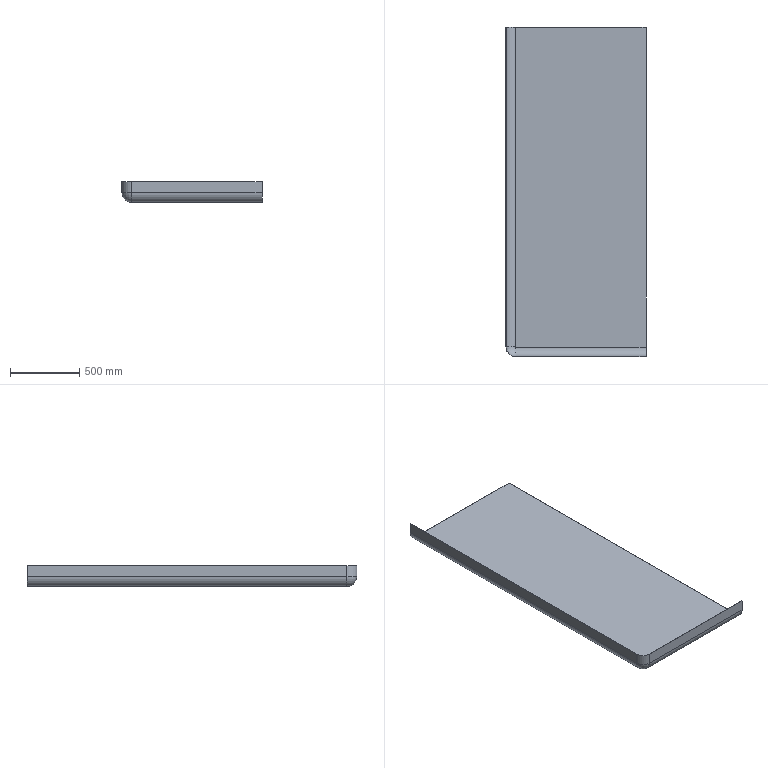Component | SolidWorks | C-SideAluminumHousingAssembly-1_C-SideAluminumCasing2-1 | 1 solid | 21 faces | box 1009.5 x 2375.5 x 149.5 mm | volume 8369304 mm3 | plane 13 | cylinder 6 | torus 2 | commonest cylinder face diameters 139 x2 133 x2 141 x1 135 x1
STEP:
#1=CARTESIAN_POINT('',(-0.2362,0.,-0.1181));
#2=VERTEX_POINT('',#1);
#3=CARTESIAN_POINT('',(-0.2362,0.,0.));
#4=VERTEX_POINT('',#3);
#5=CARTESIAN_POINT('',(-0.2362,0.,0.));
#6=DIRECTION('',(0.,0.,1.));
#7=VECTOR('',#6,39.37);
#8=LINE('',#5,#7);
#9=EDGE_CURVE('',#2,#4,#8,.T.);
#10=ORIENTED_EDGE('',*,*,#9,.F.);
#11=CARTESIAN_POINT('',(-0.2362,90.787,-0.1181));
#12=VERTEX_POINT('',#11);
#13=CARTESIAN_POINT('',(-0.2362,0.,-0.1181));
#14=DIRECTION('',(0.,1.,0.));
#15=VECTOR('',#14,39.37);
#16=LINE('',#13,#15);
#17=EDGE_CURVE('',#2,#12,#16,.T.);
#18=ORIENTED_EDGE('',*,*,#17,.T.);
#19=CARTESIAN_POINT('',(-0.2362,90.787,0.));
#20=VERTEX_POINT('',#19);
#21=CARTESIAN_POINT('',(-0.2362,90.787,0.));
#22=DIRECTION('',(0.,0.,1.));
#23=VECTOR('',#22,39.37);
#24=LINE('',#21,#23);
#25=EDGE_CURVE('',#12,#20,#24,.T.);
#26=ORIENTED_EDGE('',*,*,#25,.T.);
#27=CARTESIAN_POINT('',(-0.2362,0.,0.));
#28=DIRECTION('',(0.,1.,0.));
#29=VECTOR('',#28,39.37);
#30=LINE('',#27,#29);
#31=EDGE_CURVE('',#4,#20,#30,.T.);
#32=ORIENTED_EDGE('',*,*,#31,.F.);
#33=EDGE_LOOP('',(#10,#18,#26,#32));
#34=FACE_OUTER_BOUND('',#33,.T.);
#35=CARTESIAN_POINT('',(-0.2362,0.,0.));
#36=DIRECTION('',(-1.,0.,0.));
#37=DIRECTION('',(0.,1.,0.));
#38=AXIS2_PLACEMENT_3D('',#35,#36,#37);
#39=PLANE('',#38);
#40=ADVANCED_FACE('',(#34),#39,.F.);
#41=ORIENTED_EDGE('',*,*,#25,.F.);
#42=CARTESIAN_POINT('',(-37.244,90.787,-0.1181));
#43=VERTEX_POINT('',#42);
#44=CARTESIAN_POINT('',(-37.244,90.787,-0.1181));
#45=DIRECTION('',(-1.,0.,0.));
#46=VECTOR('',#45,39.37);
#47=LINE('',#44,#46);
#48=EDGE_CURVE('',#12,#43,#47,.T.);
#49=ORIENTED_EDGE('',*,*,#48,.T.);
#50=CARTESIAN_POINT('',(-37.244,90.787,0.));
#51=VERTEX_POINT('',#50);
#52=CARTESIAN_POINT('',(-37.244,90.787,0.));
#53=DIRECTION('',(0.,0.,1.));
#54=VECTOR('',#53,39.37);
#55=LINE('',#52,#54);
#56=EDGE_CURVE('',#43,#51,#55,.T.);
#57=ORIENTED_EDGE('',*,*,#56,.T.);
#58=CARTESIAN_POINT('',(-37.244,90.787,0.));
#59=DIRECTION('',(-1.,0.,0.));
#60=VECTOR('',#59,39.37);
#61=LINE('',#58,#60);
#62=EDGE_CURVE('',#20,#51,#61,.T.);
#63=ORIENTED_EDGE('',*,*,#62,.F.);
#64=EDGE_LOOP('',(#41,#49,#57,#63));
#65=FACE_OUTER_BOUND('',#64,.T.);
#66=CARTESIAN_POINT('',(-37.244,90.787,0.));
#67=DIRECTION('',(0.,-1.,0.));
#68=DIRECTION('',(-1.,0.,0.));
#69=AXIS2_PLACEMENT_3D('',#66,#67,#68);
#70=PLANE('',#69);
#71=ADVANCED_FACE('',(#65),#70,.F.);
#72=CARTESIAN_POINT('',(-37.244,0.03937,0.));
#73=VERTEX_POINT('',#72);
#74=CARTESIAN_POINT('',(-37.244,0.,0.));
#75=DIRECTION('',(0.,-1.,0.));
#76=VECTOR('',#75,39.37);
#77=LINE('',#74,#76);
#78=EDGE_CURVE('',#51,#73,#77,.T.);
#79=ORIENTED_EDGE('',*,*,#78,.T.);
#80=CARTESIAN_POINT('',(-37.205,0.,0.));
#81=VERTEX_POINT('',#80);
#82=CARTESIAN_POINT('',(-37.205,0.03937,0.));
#83=DIRECTION('',(0.,0.,1.));
#84=DIRECTION('',(-1.,0.,0.));
#85=AXIS2_PLACEMENT_3D('',#82,#83,#84);
#86=CIRCLE('',#85,0.03937);
#87=EDGE_CURVE('',#73,#81,#86,.T.);
#88=ORIENTED_EDGE('',*,*,#87,.T.);
#89=CARTESIAN_POINT('',(-37.244,0.,0.));
#90=DIRECTION('',(1.,0.,0.));
#91=VECTOR('',#90,39.37);
#92=LINE('',#89,#91);
#93=EDGE_CURVE('',#81,#4,#92,.T.);
#94=ORIENTED_EDGE('',*,*,#93,.T.);
#95=ORIENTED_EDGE('',*,*,#31,.T.);
#96=ORIENTED_EDGE('',*,*,#62,.T.);
#97=EDGE_LOOP('',(#79,#88,#94,#95,#96));
#98=FACE_OUTER_BOUND('',#97,.T.);
#99=CARTESIAN_POINT('',(-37.244,0.,0.));
#100=DIRECTION('',(0.,0.,-1.));
#101=DIRECTION('',(-1.,0.,0.));
#102=AXIS2_PLACEMENT_3D('',#99,#100,#101);
#103=PLANE('',#102);
#104=ADVANCED_FACE('',(#98),#103,.F.);
#105=CARTESIAN_POINT('',(-37.205,0.,-0.1181));
#106=VERTEX_POINT('',#105);
#107=CARTESIAN_POINT('',(-37.244,0.,-0.1181));
#108=DIRECTION('',(1.,0.,0.));
#109=VECTOR('',#108,39.37);
#110=LINE('',#107,#109);
#111=EDGE_CURVE('',#106,#2,#110,.T.);
#112=ORIENTED_EDGE('',*,*,#111,.F.);
#113=CARTESIAN_POINT('',(-37.244,0.03937,-0.1181));
#114=VERTEX_POINT('',#113);
#115=CARTESIAN_POINT('',(-37.205,0.03937,-0.1181));
#116=DIRECTION('',(0.,0.,-1.));
#117=DIRECTION('',(-1.,0.,0.));
#118=AXIS2_PLACEMENT_3D('',#115,#116,#117);
#119=CIRCLE('',#118,0.03937);
#120=EDGE_CURVE('',#106,#114,#119,.T.);
#121=ORIENTED_EDGE('',*,*,#120,.T.);
#122=CARTESIAN_POINT('',(-37.244,0.,-0.1181));
#123=DIRECTION('',(0.,-1.,0.));
#124=VECTOR('',#123,39.37);
#125=LINE('',#122,#124);
#126=EDGE_CURVE('',#43,#114,#125,.T.);
#127=ORIENTED_EDGE('',*,*,#126,.F.);
#128=ORIENTED_EDGE('',*,*,#48,.F.);
#129=ORIENTED_EDGE('',*,*,#17,.F.);
#130=EDGE_LOOP('',(#112,#121,#127,#128,#129));
#131=FACE_OUTER_BOUND('',#130,.T.);
#132=CARTESIAN_POINT('',(-37.244,0.,-0.1181));
#133=DIRECTION('',(0.,0.,-1.));
#134=DIRECTION('',(-1.,0.,0.));
#135=AXIS2_PLACEMENT_3D('',#132,#133,#134);
#136=PLANE('',#135);
#137=ADVANCED_FACE('',(#131),#136,.T.);
#138=CARTESIAN_POINT('',(-0.2362,-2.618,2.618));
#139=VERTEX_POINT('',#138);
#140=CARTESIAN_POINT('',(-0.2362,0.,2.618));
#141=DIRECTION('',(1.,0.,0.));
#142=DIRECTION('',(0.,0.,-1.));
#143=AXIS2_PLACEMENT_3D('',#140,#141,#142);
#144=CIRCLE('',#143,2.618);
#145=EDGE_CURVE('',#139,#4,#144,.T.);
#146=ORIENTED_EDGE('',*,*,#145,.F.);
#147=CARTESIAN_POINT('',(-0.2362,-2.736,2.618));
#148=VERTEX_POINT('',#147);
#149=CARTESIAN_POINT('',(-0.2362,-2.618,2.618));
#150=DIRECTION('',(0.,-1.,-0.));
#151=VECTOR('',#150,39.37);
#152=LINE('',#149,#151);
#153=EDGE_CURVE('',#139,#148,#152,.T.);
#154=ORIENTED_EDGE('',*,*,#153,.T.);
#155=CARTESIAN_POINT('',(-0.2362,0.,2.618));
#156=DIRECTION('',(1.,0.,0.));
#157=DIRECTION('',(0.,0.,-1.));
#158=AXIS2_PLACEMENT_3D('',#155,#156,#157);
#159=CIRCLE('',#158,2.736);
#160=EDGE_CURVE('',#148,#2,#159,.T.);
#161=ORIENTED_EDGE('',*,*,#160,.T.);
#162=ORIENTED_EDGE('',*,*,#9,.T.);
#163=EDGE_LOOP('',(#146,#154,#161,#162));
#164=FACE_OUTER_BOUND('',#163,.T.);
#165=CARTESIAN_POINT('',(-0.2362,0.,2.618));
#166=DIRECTION('',(-1.,0.,0.));
#167=DIRECTION('',(0.,0.,1.));
#168=AXIS2_PLACEMENT_3D('',#165,#166,#167);
#169=PLANE('',#168);
#170=ADVANCED_FACE('',(#164),#169,.F.);
#171=ORIENTED_EDGE('',*,*,#111,.T.);
#172=ORIENTED_EDGE('',*,*,#160,.F.);
#173=CARTESIAN_POINT('',(-37.205,-2.736,2.618));
#174=VERTEX_POINT('',#173);
#175=CARTESIAN_POINT('',(-37.205,-2.736,2.618));
#176=DIRECTION('',(-1.,0.,0.));
#177=VECTOR('',#176,39.37);
#178=LINE('',#175,#177);
#179=EDGE_CURVE('',#148,#174,#178,.T.);
#180=ORIENTED_EDGE('',*,*,#179,.T.);
#181=CARTESIAN_POINT('',(-37.205,0.,2.618));
#182=DIRECTION('',(-1.,0.,0.));
#183=DIRECTION('',(0.,0.,-1.));
#184=AXIS2_PLACEMENT_3D('',#181,#182,#183);
#185=CIRCLE('',#184,2.736);
#186=EDGE_CURVE('',#106,#174,#185,.T.);
#187=ORIENTED_EDGE('',*,*,#186,.F.);
#188=EDGE_LOOP('',(#171,#172,#180,#187));
#189=FACE_OUTER_BOUND('',#188,.T.);
#190=CARTESIAN_POINT('',(-0.2362,0.,2.618));
#191=DIRECTION('',(1.,0.,0.));
#192=DIRECTION('',(0.,-1.,-0.));
#193=AXIS2_PLACEMENT_3D('',#190,#191,#192);
#194=CYLINDRICAL_SURFACE('',#193,2.736);
#195=ADVANCED_FACE('',(#189),#194,.T.);
#196=ORIENTED_EDGE('',*,*,#93,.F.);
#197=CARTESIAN_POINT('',(-37.205,-2.618,2.618));
#198=VERTEX_POINT('',#197);
#199=CARTESIAN_POINT('',(-37.205,0.,2.618));
#200=DIRECTION('',(-1.,0.,0.));
#201=DIRECTION('',(0.,0.,-1.));
#202=AXIS2_PLACEMENT_3D('',#199,#200,#201);
#203=CIRCLE('',#202,2.618);
#204=EDGE_CURVE('',#81,#198,#203,.T.);
#205=ORIENTED_EDGE('',*,*,#204,.T.);
#206=CARTESIAN_POINT('',(-37.205,-2.618,2.618));
#207=DIRECTION('',(1.,0.,0.));
#208=VECTOR('',#207,39.37);
#209=LINE('',#206,#208);
#210=EDGE_CURVE('',#198,#139,#209,.T.);
#211=ORIENTED_EDGE('',*,*,#210,.T.);
#212=ORIENTED_EDGE('',*,*,#145,.T.);
#213=EDGE_LOOP('',(#196,#205,#211,#212));
#214=FACE_OUTER_BOUND('',#213,.T.);
#215=CARTESIAN_POINT('',(-0.2362,0.,2.618));
#216=DIRECTION('',(1.,0.,0.));
#217=DIRECTION('',(0.,-1.,-0.));
#218=AXIS2_PLACEMENT_3D('',#215,#216,#217);
#219=CYLINDRICAL_SURFACE('',#218,2.618);
#220=ADVANCED_FACE('',(#214),#219,.F.);
#221=ORIENTED_EDGE('',*,*,#153,.F.);
#222=CARTESIAN_POINT('',(-0.2362,-2.618,5.768));
#223=VERTEX_POINT('',#222);
#224=CARTESIAN_POINT('',(-0.2362,-2.618,5.768));
#225=DIRECTION('',(0.,-0.,1.));
#226=VECTOR('',#225,39.37);
#227=LINE('',#224,#226);
#228=EDGE_CURVE('',#139,#223,#227,.T.);
#229=ORIENTED_EDGE('',*,*,#228,.T.);
#230=CARTESIAN_POINT('',(-0.2362,-2.736,5.768));
#231=VERTEX_POINT('',#230);
#232=CARTESIAN_POINT('',(-0.2362,-2.736,5.768));
#233=DIRECTION('',(0.,1.,0.));
#234=VECTOR('',#233,39.37);
#235=LINE('',#232,#234);
#236=EDGE_CURVE('',#231,#223,#235,.T.);
#237=ORIENTED_EDGE('',*,*,#236,.F.);
#238=CARTESIAN_POINT('',(-0.2362,-2.736,-0.));
#239=DIRECTION('',(0.,-0.,1.));
#240=VECTOR('',#239,39.37);
#241=LINE('',#238,#240);
#242=EDGE_CURVE('',#148,#231,#241,.T.);
#243=ORIENTED_EDGE('',*,*,#242,.F.);
#244=EDGE_LOOP('',(#221,#229,#237,#243));
#245=FACE_OUTER_BOUND('',#244,.T.);
#246=CARTESIAN_POINT('',(-0.2362,-2.736,5.768));
#247=DIRECTION('',(-1.,0.,0.));
#248=DIRECTION('',(0.,0.,1.));
#249=AXIS2_PLACEMENT_3D('',#246,#247,#248);
#250=PLANE('',#249);
#251=ADVANCED_FACE('',(#245),#250,.F.);
#252=ORIENTED_EDGE('',*,*,#179,.F.);
#253=ORIENTED_EDGE('',*,*,#242,.T.);
#254=CARTESIAN_POINT('',(-37.205,-2.736,5.768));
#255=VERTEX_POINT('',#254);
#256=CARTESIAN_POINT('',(-37.244,-2.736,5.768));
#257=DIRECTION('',(-1.,0.,0.));
#258=VECTOR('',#257,39.37);
#259=LINE('',#256,#258);
#260=EDGE_CURVE('',#231,#255,#259,.T.);
#261=ORIENTED_EDGE('',*,*,#260,.T.);
#262=CARTESIAN_POINT('',(-37.205,-2.736,-0.));
#263=DIRECTION('',(0.,0.,-1.));
#264=VECTOR('',#263,39.37);
#265=LINE('',#262,#264);
#266=EDGE_CURVE('',#255,#174,#265,.T.);
#267=ORIENTED_EDGE('',*,*,#266,.T.);
#268=EDGE_LOOP('',(#252,#253,#261,#267));
#269=FACE_OUTER_BOUND('',#268,.T.);
#270=CARTESIAN_POINT('',(-37.244,-2.736,-0.));
#271=DIRECTION('',(0.,1.,0.));
#272=DIRECTION('',(0.,-0.,1.));
#273=AXIS2_PLACEMENT_3D('',#270,#271,#272);
#274=PLANE('',#273);
#275=ADVANCED_FACE('',(#269),#274,.F.);
#276=ORIENTED_EDGE('',*,*,#228,.F.);
#277=ORIENTED_EDGE('',*,*,#210,.F.);
#278=CARTESIAN_POINT('',(-37.205,-2.618,5.768));
#279=VERTEX_POINT('',#278);
#280=CARTESIAN_POINT('',(-37.205,-2.618,0.));
#281=DIRECTION('',(0.,0.,-1.));
#282=VECTOR('',#281,39.37);
#283=LINE('',#280,#282);
#284=EDGE_CURVE('',#279,#198,#283,.T.);
#285=ORIENTED_EDGE('',*,*,#284,.F.);
#286=CARTESIAN_POINT('',(-37.205,-2.618,5.768));
#287=DIRECTION('',(-1.,0.,0.));
#288=VECTOR('',#287,39.37);
#289=LINE('',#286,#288);
#290=EDGE_CURVE('',#223,#279,#289,.T.);
#291=ORIENTED_EDGE('',*,*,#290,.F.);
#292=EDGE_LOOP('',(#276,#277,#285,#291));
#293=FACE_OUTER_BOUND('',#292,.T.);
#294=CARTESIAN_POINT('',(-37.244,-2.618,0.));
#295=DIRECTION('',(0.,1.,0.));
#296=DIRECTION('',(0.,-0.,1.));
#297=AXIS2_PLACEMENT_3D('',#294,#295,#296);
#298=PLANE('',#297);
#299=ADVANCED_FACE('',(#293),#298,.T.);
#300=ORIENTED_EDGE('',*,*,#290,.T.);
#301=CARTESIAN_POINT('',(-39.862,0.03937,5.768));
#302=VERTEX_POINT('',#301);
#303=CARTESIAN_POINT('',(-37.205,0.03937,5.768));
#304=DIRECTION('',(0.,0.,1.));
#305=DIRECTION('',(-1.,-0.,0.));
#306=AXIS2_PLACEMENT_3D('',#303,#304,#305);
#307=CIRCLE('',#306,2.657);
#308=EDGE_CURVE('',#302,#279,#307,.T.);
#309=ORIENTED_EDGE('',*,*,#308,.F.);
#310=CARTESIAN_POINT('',(-39.862,90.787,5.768));
#311=VERTEX_POINT('',#310);
#312=CARTESIAN_POINT('',(-39.862,90.787,5.768));
#313=DIRECTION('',(0.,1.,0.));
#314=VECTOR('',#313,39.37);
#315=LINE('',#312,#314);
#316=EDGE_CURVE('',#302,#311,#315,.T.);
#317=ORIENTED_EDGE('',*,*,#316,.T.);
#318=CARTESIAN_POINT('',(-39.98,90.787,5.768));
#319=VERTEX_POINT('',#318);
#320=CARTESIAN_POINT('',(-39.98,90.787,5.768));
#321=DIRECTION('',(1.,0.,0.));
#322=VECTOR('',#321,39.37);
#323=LINE('',#320,#322);
#324=EDGE_CURVE('',#319,#311,#323,.T.);
#325=ORIENTED_EDGE('',*,*,#324,.F.);
#326=CARTESIAN_POINT('',(-39.98,0.03937,5.768));
#327=VERTEX_POINT('',#326);
#328=CARTESIAN_POINT('',(-39.98,0.,5.768));
#329=DIRECTION('',(0.,1.,0.));
#330=VECTOR('',#329,39.37);
#331=LINE('',#328,#330);
#332=EDGE_CURVE('',#327,#319,#331,.T.);
#333=ORIENTED_EDGE('',*,*,#332,.F.);
#334=CARTESIAN_POINT('',(-37.205,0.03937,5.768));
#335=DIRECTION('',(0.,0.,1.));
#336=DIRECTION('',(-1.,-0.,0.));
#337=AXIS2_PLACEMENT_3D('',#334,#335,#336);
#338=CIRCLE('',#337,2.776);
#339=EDGE_CURVE('',#327,#255,#338,.T.);
#340=ORIENTED_EDGE('',*,*,#339,.T.);
#341=ORIENTED_EDGE('',*,*,#260,.F.);
#342=ORIENTED_EDGE('',*,*,#236,.T.);
#343=EDGE_LOOP('',(#300,#309,#317,#325,#333,#340,#341,#342));
#344=FACE_OUTER_BOUND('',#343,.T.);
#345=CARTESIAN_POINT('',(-37.205,-2.736,5.768));
#346=DIRECTION('',(0.,0.,-1.));
#347=DIRECTION('',(0.,1.,0.));
#348=AXIS2_PLACEMENT_3D('',#345,#346,#347);
#349=PLANE('',#348);
#350=ADVANCED_FACE('',(#344),#349,.F.);
#351=CARTESIAN_POINT('',(-39.862,90.787,2.618));
#352=VERTEX_POINT('',#351);
#353=CARTESIAN_POINT('',(-39.98,90.787,2.618));
#354=VERTEX_POINT('',#353);
#355=CARTESIAN_POINT('',(-39.98,90.787,2.618));
#356=DIRECTION('',(-1.,0.,-0.));
#357=VECTOR('',#356,39.37);
#358=LINE('',#355,#357);
#359=EDGE_CURVE('',#352,#354,#358,.T.);
#360=ORIENTED_EDGE('',*,*,#359,.F.);
#361=CARTESIAN_POINT('',(-37.244,90.787,2.618));
#362=DIRECTION('',(0.,1.,0.));
#363=DIRECTION('',(0.,0.,-1.));
#364=AXIS2_PLACEMENT_3D('',#361,#362,#363);
#365=CIRCLE('',#364,2.618);
#366=EDGE_CURVE('',#51,#352,#365,.T.);
#367=ORIENTED_EDGE('',*,*,#366,.F.);
#368=ORIENTED_EDGE('',*,*,#56,.F.);
#369=CARTESIAN_POINT('',(-37.244,90.787,2.618));
#370=DIRECTION('',(0.,1.,0.));
#371=DIRECTION('',(0.,0.,-1.));
#372=AXIS2_PLACEMENT_3D('',#369,#370,#371);
#373=CIRCLE('',#372,2.736);
#374=EDGE_CURVE('',#43,#354,#373,.T.);
#375=ORIENTED_EDGE('',*,*,#374,.T.);
#376=EDGE_LOOP('',(#360,#367,#368,#375));
#377=FACE_OUTER_BOUND('',#376,.T.);
#378=CARTESIAN_POINT('',(-37.244,90.787,2.618));
#379=DIRECTION('',(0.,1.,0.));
#380=DIRECTION('',(0.,0.,1.));
#381=AXIS2_PLACEMENT_3D('',#378,#379,#380);
#382=PLANE('',#381);
#383=ADVANCED_FACE('',(#377),#382,.T.);
#384=ORIENTED_EDGE('',*,*,#126,.T.);
#385=CARTESIAN_POINT('',(-39.98,0.03937,2.618));
#386=VERTEX_POINT('',#385);
#387=CARTESIAN_POINT('',(-37.244,0.03937,2.618));
#388=DIRECTION('',(0.,-1.,0.));
#389=DIRECTION('',(0.,0.,-1.));
#390=AXIS2_PLACEMENT_3D('',#387,#388,#389);
#391=CIRCLE('',#390,2.736);
#392=EDGE_CURVE('',#386,#114,#391,.T.);
#393=ORIENTED_EDGE('',*,*,#392,.F.);
#394=CARTESIAN_POINT('',(-39.98,90.787,2.618));
#395=DIRECTION('',(0.,1.,0.));
#396=VECTOR('',#395,39.37);
#397=LINE('',#394,#396);
#398=EDGE_CURVE('',#386,#354,#397,.T.);
#399=ORIENTED_EDGE('',*,*,#398,.T.);
#400=ORIENTED_EDGE('',*,*,#374,.F.);
#401=EDGE_LOOP('',(#384,#393,#399,#400));
#402=FACE_OUTER_BOUND('',#401,.T.);
#403=CARTESIAN_POINT('',(-37.244,0.03937,2.618));
#404=DIRECTION('',(0.,-1.,0.));
#405=DIRECTION('',(-1.,0.,-0.));
#406=AXIS2_PLACEMENT_3D('',#403,#404,#405);
#407=CYLINDRICAL_SURFACE('',#406,2.736);
#408=ADVANCED_FACE('',(#402),#407,.T.);
#409=ORIENTED_EDGE('',*,*,#78,.F.);
#410=ORIENTED_EDGE('',*,*,#366,.T.);
#411=CARTESIAN_POINT('',(-39.862,0.03937,2.618));
#412=VERTEX_POINT('',#411);
#413=CARTESIAN_POINT('',(-39.862,90.787,2.618));
#414=DIRECTION('',(0.,-1.,0.));
#415=VECTOR('',#414,39.37);
#416=LINE('',#413,#415);
#417=EDGE_CURVE('',#352,#412,#416,.T.);
#418=ORIENTED_EDGE('',*,*,#417,.T.);
#419=CARTESIAN_POINT('',(-37.244,0.03937,2.618));
#420=DIRECTION('',(0.,-1.,0.));
#421=DIRECTION('',(0.,0.,-1.));
#422=AXIS2_PLACEMENT_3D('',#419,#420,#421);
#423=CIRCLE('',#422,2.618);
#424=EDGE_CURVE('',#412,#73,#423,.T.);
#425=ORIENTED_EDGE('',*,*,#424,.T.);
#426=EDGE_LOOP('',(#409,#410,#418,#425));
#427=FACE_OUTER_BOUND('',#426,.T.);
#428=CARTESIAN_POINT('',(-37.244,0.03937,2.618));
#429=DIRECTION('',(0.,-1.,0.));
#430=DIRECTION('',(-1.,0.,-0.));
#431=AXIS2_PLACEMENT_3D('',#428,#429,#430);
#432=CYLINDRICAL_SURFACE('',#431,2.618);
#433=ADVANCED_FACE('',(#427),#432,.F.);
#434=ORIENTED_EDGE('',*,*,#359,.T.);
#435=CARTESIAN_POINT('',(-39.98,90.787,-0.));
#436=DIRECTION('',(0.,0.,-1.));
#437=VECTOR('',#436,39.37);
#438=LINE('',#435,#437);
#439=EDGE_CURVE('',#319,#354,#438,.T.);
#440=ORIENTED_EDGE('',*,*,#439,.F.);
#441=ORIENTED_EDGE('',*,*,#324,.T.);
#442=CARTESIAN_POINT('',(-39.862,90.787,0.));
#443=DIRECTION('',(0.,0.,-1.));
#444=VECTOR('',#443,39.37);
#445=LINE('',#442,#444);
#446=EDGE_CURVE('',#311,#352,#445,.T.);
#447=ORIENTED_EDGE('',*,*,#446,.T.);
#448=EDGE_LOOP('',(#434,#440,#441,#447));
#449=FACE_OUTER_BOUND('',#448,.T.);
#450=CARTESIAN_POINT('',(-39.98,90.787,-0.));
#451=DIRECTION('',(0.,-1.,0.));
#452=DIRECTION('',(0.,0.,-1.));
#453=AXIS2_PLACEMENT_3D('',#450,#451,#452);
#454=PLANE('',#453);
#455=ADVANCED_FACE('',(#449),#454,.F.);
#456=ORIENTED_EDGE('',*,*,#398,.F.);
#457=CARTESIAN_POINT('',(-39.98,0.03937,-0.));
#458=DIRECTION('',(-0.,0.,1.));
#459=VECTOR('',#458,39.37);
#460=LINE('',#457,#459);
#461=EDGE_CURVE('',#386,#327,#460,.T.);
#462=ORIENTED_EDGE('',*,*,#461,.T.);
#463=ORIENTED_EDGE('',*,*,#332,.T.);
#464=ORIENTED_EDGE('',*,*,#439,.T.);
#465=EDGE_LOOP('',(#456,#462,#463,#464));
#466=FACE_OUTER_BOUND('',#465,.T.);
#467=CARTESIAN_POINT('',(-39.98,0.,-0.));
#468=DIRECTION('',(1.,0.,0.));
#469=DIRECTION('',(0.,0.,-1.));
#470=AXIS2_PLACEMENT_3D('',#467,#468,#469);
#471=PLANE('',#470);
#472=ADVANCED_FACE('',(#466),#471,.F.);
#473=CARTESIAN_POINT('',(-39.862,0.03937,5.768));
#474=DIRECTION('',(-0.,0.,1.));
#475=VECTOR('',#474,39.37);
#476=LINE('',#473,#475);
#477=EDGE_CURVE('',#412,#302,#476,.T.);
#478=ORIENTED_EDGE('',*,*,#477,.F.);
#479=ORIENTED_EDGE('',*,*,#417,.F.);
#480=ORIENTED_EDGE('',*,*,#446,.F.);
#481=ORIENTED_EDGE('',*,*,#316,.F.);
#482=EDGE_LOOP('',(#478,#479,#480,#481));
#483=FACE_OUTER_BOUND('',#482,.T.);
#484=CARTESIAN_POINT('',(-39.862,0.,0.));
#485=DIRECTION('',(1.,0.,0.));
#486=DIRECTION('',(0.,0.,-1.));
#487=AXIS2_PLACEMENT_3D('',#484,#485,#486);
#488=PLANE('',#487);
#489=ADVANCED_FACE('',(#483),#488,.T.);
#490=ORIENTED_EDGE('',*,*,#87,.F.);
#491=ORIENTED_EDGE('',*,*,#424,.F.);
#492=CARTESIAN_POINT('',(-37.205,0.03937,2.618));
#493=DIRECTION('',(0.,0.,1.));
#494=DIRECTION('',(-1.,-0.,0.));
#495=AXIS2_PLACEMENT_3D('',#492,#493,#494);
#496=CIRCLE('',#495,2.657);
#497=EDGE_CURVE('',#412,#198,#496,.T.);
#498=ORIENTED_EDGE('',*,*,#497,.T.);
#499=ORIENTED_EDGE('',*,*,#204,.F.);
#500=EDGE_LOOP('',(#490,#491,#498,#499));
#501=FACE_OUTER_BOUND('',#500,.T.);
#502=CARTESIAN_POINT('',(-37.205,0.03937,2.618));
#503=DIRECTION('',(0.,0.,1.));
#504=DIRECTION('',(1.,0.,0.));
#505=AXIS2_PLACEMENT_3D('',#502,#503,#504);
#506=TOROIDAL_SURFACE('',#505,0.03937,2.618);
#507=ADVANCED_FACE('',(#501),#506,.F.);
#508=CARTESIAN_POINT('',(-37.205,0.03937,2.618));
#509=DIRECTION('',(0.,0.,1.));
#510=DIRECTION('',(-1.,-0.,0.));
#511=AXIS2_PLACEMENT_3D('',#508,#509,#510);
#512=CIRCLE('',#511,2.776);
#513=EDGE_CURVE('',#386,#174,#512,.T.);
#514=ORIENTED_EDGE('',*,*,#513,.F.);
#515=ORIENTED_EDGE('',*,*,#392,.T.);
#516=ORIENTED_EDGE('',*,*,#120,.F.);
#517=ORIENTED_EDGE('',*,*,#186,.T.);
#518=EDGE_LOOP('',(#514,#515,#516,#517));
#519=FACE_OUTER_BOUND('',#518,.T.);
#520=CARTESIAN_POINT('',(-37.205,0.03937,2.618));
#521=DIRECTION('',(0.,0.,1.));
#522=DIRECTION('',(1.,0.,0.));
#523=AXIS2_PLACEMENT_3D('',#520,#521,#522);
#524=TOROIDAL_SURFACE('',#523,0.03937,2.736);
#525=ADVANCED_FACE('',(#519),#524,.T.);
#526=ORIENTED_EDGE('',*,*,#339,.F.);
#527=ORIENTED_EDGE('',*,*,#461,.F.);
#528=ORIENTED_EDGE('',*,*,#513,.T.);
#529=ORIENTED_EDGE('',*,*,#266,.F.);
#530=EDGE_LOOP('',(#526,#527,#528,#529));
#531=FACE_OUTER_BOUND('',#530,.T.);
#532=CARTESIAN_POINT('',(-37.205,0.03937,2.618));
#533=DIRECTION('',(0.,0.,1.));
#534=DIRECTION('',(1.,0.,0.));
#535=AXIS2_PLACEMENT_3D('',#532,#533,#534);
#536=CYLINDRICAL_SURFACE('',#535,2.776);
#537=ADVANCED_FACE('',(#531),#536,.T.);
#538=ORIENTED_EDGE('',*,*,#497,.F.);
#539=ORIENTED_EDGE('',*,*,#477,.T.);
#540=ORIENTED_EDGE('',*,*,#308,.T.);
#541=ORIENTED_EDGE('',*,*,#284,.T.);
#542=EDGE_LOOP('',(#538,#539,#540,#541));
#543=FACE_OUTER_BOUND('',#542,.T.);
#544=CARTESIAN_POINT('',(-37.205,0.03937,2.618));
#545=DIRECTION('',(0.,0.,1.));
#546=DIRECTION('',(1.,0.,0.));
#547=AXIS2_PLACEMENT_3D('',#544,#545,#546);
#548=CYLINDRICAL_SURFACE('',#547,2.657);
#549=ADVANCED_FACE('',(#543),#548,.F.);
#550=CLOSED_SHELL('',(#40,#71,#104,#137,#170,#195,#220,#251,#275,#299,#350,#383,#408,#433,#455,#472,#489,#507,#525,#537,#549));
#551=MANIFOLD_SOLID_BREP('',#550);
#552=CARTESIAN_POINT('',(0.,0.,0.));
#553=DIRECTION('',(0.,0.,1.));
#554=DIRECTION('',(1.,0.,0.));
#555=AXIS2_PLACEMENT_3D('',#552,#553,#554);
#556=(LENGTH_UNIT()NAMED_UNIT(*)SI_UNIT($,.METRE.));
#557=LENGTH_MEASURE_WITH_UNIT(LENGTH_MEASURE(0.0254),#556);
#558=DIMENSIONAL_EXPONENTS(1.,0.,0.,0.,0.,0.,0.);
#559=(CONVERSION_BASED_UNIT('',#557)LENGTH_UNIT()NAMED_UNIT(#558));
#560=UNCERTAINTY_MEASURE_WITH_UNIT(LENGTH_MEASURE(0.00001),#559,'','');
#561=(NAMED_UNIT(*)PLANE_ANGLE_UNIT()SI_UNIT($,.RADIAN.));
#562=(NAMED_UNIT(*)SI_UNIT($,.STERADIAN.)SOLID_ANGLE_UNIT());
#563=(GEOMETRIC_REPRESENTATION_CONTEXT(3)GLOBAL_UNCERTAINTY_ASSIGNED_CONTEXT((#560))GLOBAL_UNIT_ASSIGNED_CONTEXT((#559,#561,#562))REPRESENTATION_CONTEXT('',''));
#564=ADVANCED_BREP_SHAPE_REPRESENTATION('',(#551,#555),#563);
#565=COLOUR_RGB('',0.7922,0.8196,0.9333);
#566=FILL_AREA_STYLE_COLOUR('',#565);
#567=FILL_AREA_STYLE('',(#566));
#568=SURFACE_STYLE_FILL_AREA(#567);
#569=SURFACE_SIDE_STYLE('',(#568));
#570=SURFACE_STYLE_USAGE(.BOTH.,#569);
#571=PRESENTATION_STYLE_ASSIGNMENT((#570));
#572=STYLED_ITEM('',(#571),#551);
#573=(LENGTH_UNIT()NAMED_UNIT(*)SI_UNIT($,.METRE.));
#574=LENGTH_MEASURE_WITH_UNIT(LENGTH_MEASURE(0.0254),#573);
#575=DIMENSIONAL_EXPONENTS(1.,0.,0.,0.,0.,0.,0.);
#576=(CONVERSION_BASED_UNIT('',#574)LENGTH_UNIT()NAMED_UNIT(#575));
#577=UNCERTAINTY_MEASURE_WITH_UNIT(LENGTH_MEASURE(0.00001),#576,'','');
#578=(NAMED_UNIT(*)PLANE_ANGLE_UNIT()SI_UNIT($,.RADIAN.));
#579=(NAMED_UNIT(*)SI_UNIT($,.STERADIAN.)SOLID_ANGLE_UNIT());
#580=(GEOMETRIC_REPRESENTATION_CONTEXT(3)GLOBAL_UNCERTAINTY_ASSIGNED_CONTEXT((#577))GLOBAL_UNIT_ASSIGNED_CONTEXT((#576,#578,#579))REPRESENTATION_CONTEXT('',''));
#581=MECHANICAL_DESIGN_GEOMETRIC_PRESENTATION_REPRESENTATION('',(#572),#580);
#582=PRESENTATION_LAYER_ASSIGNMENT('','',(#572));